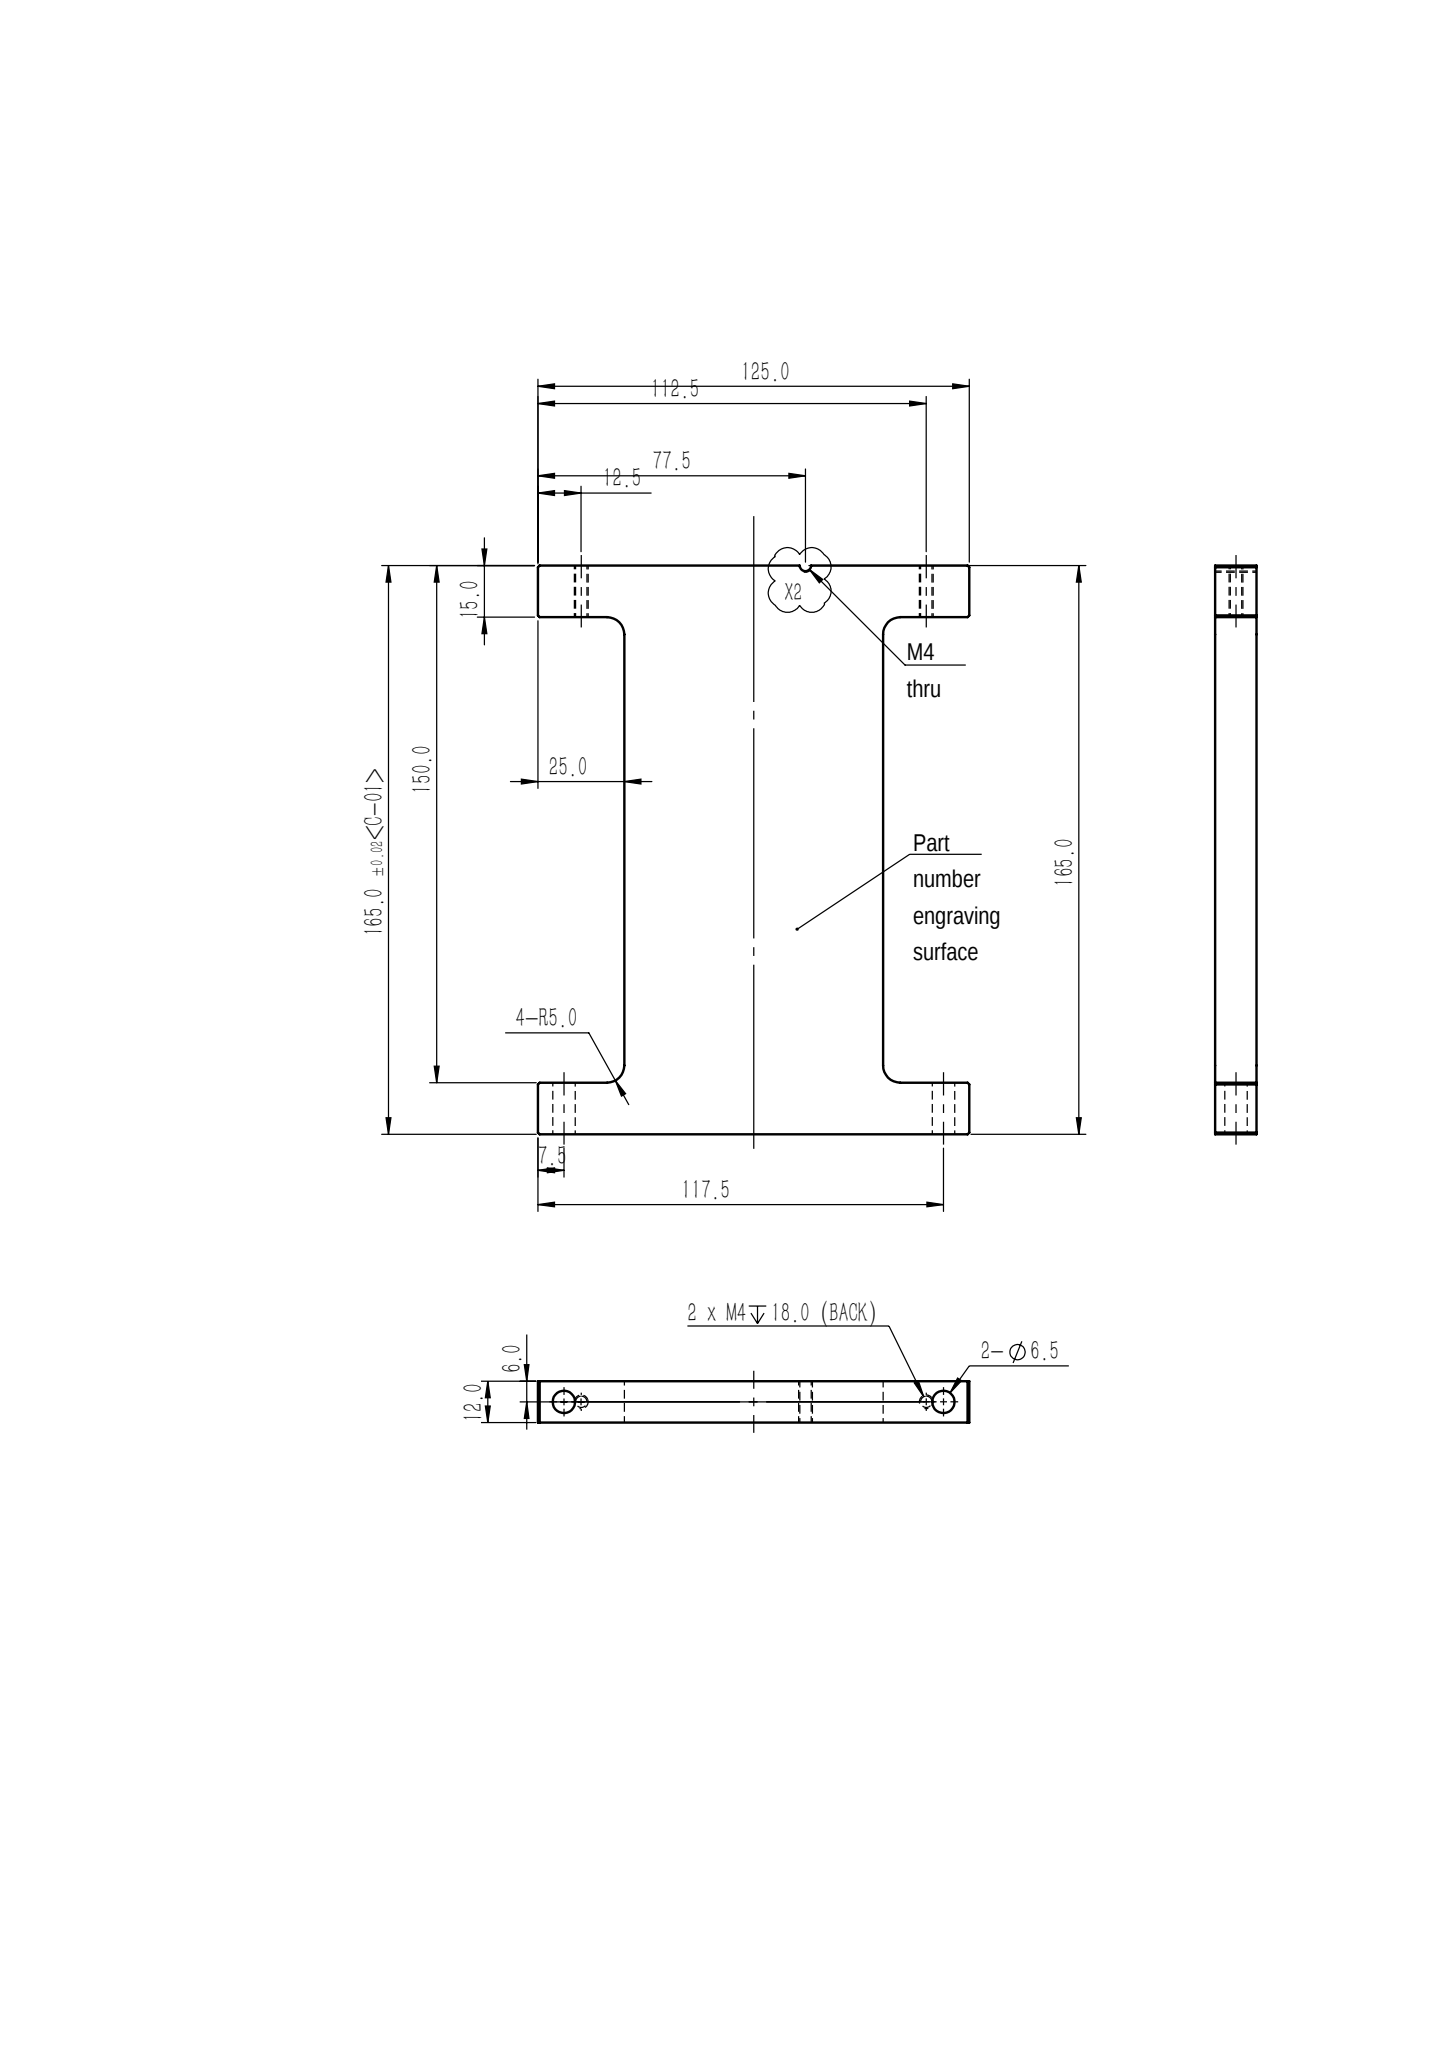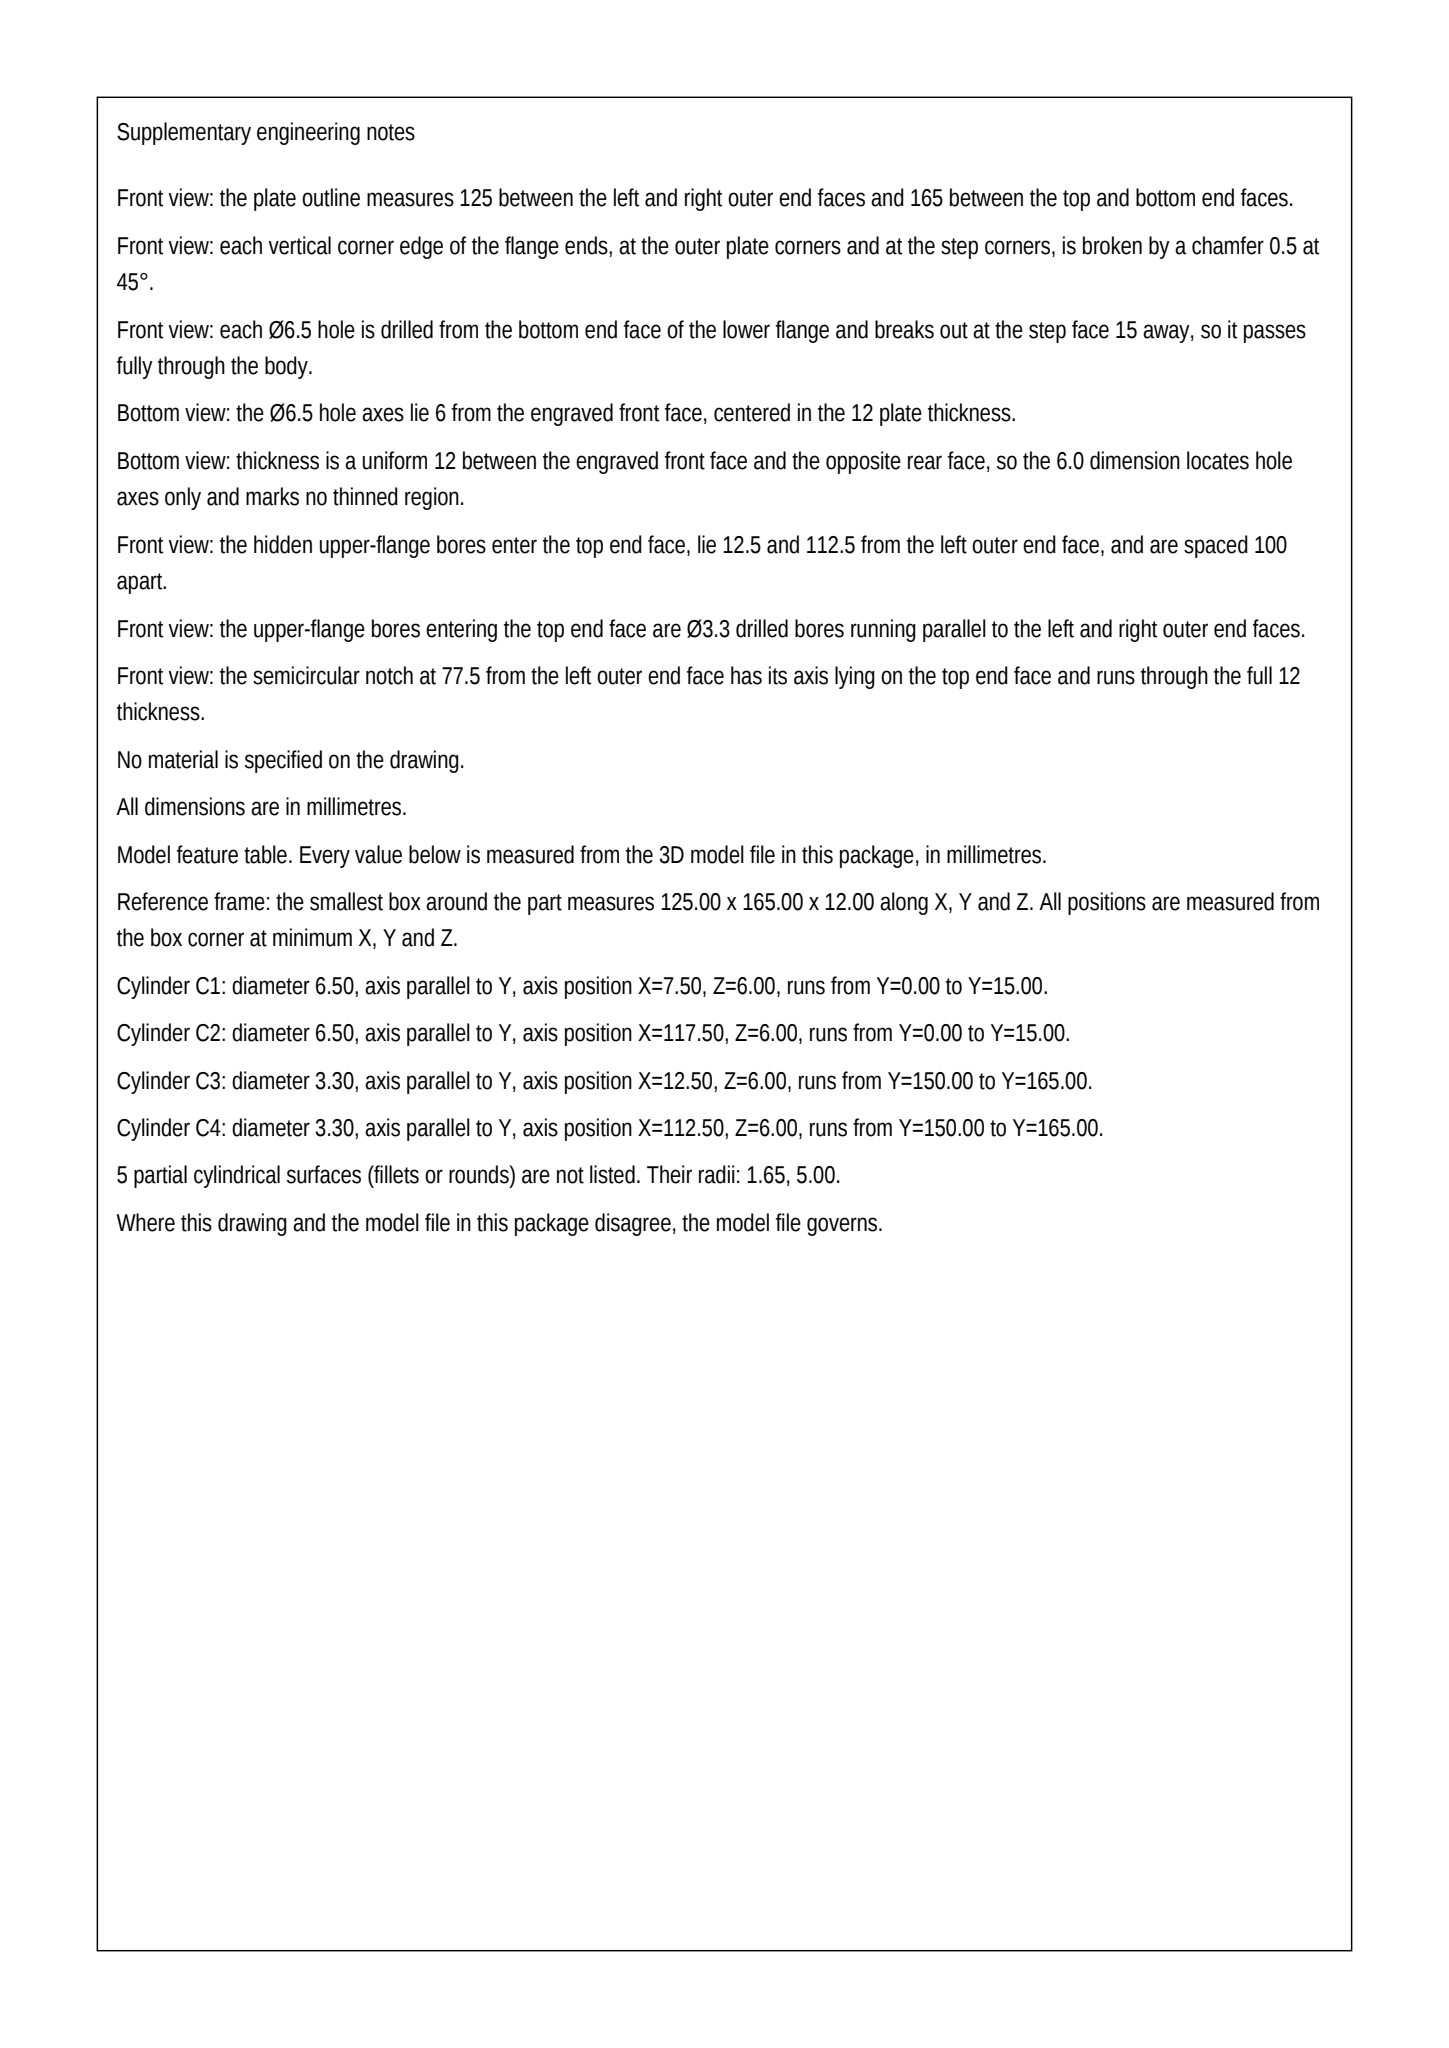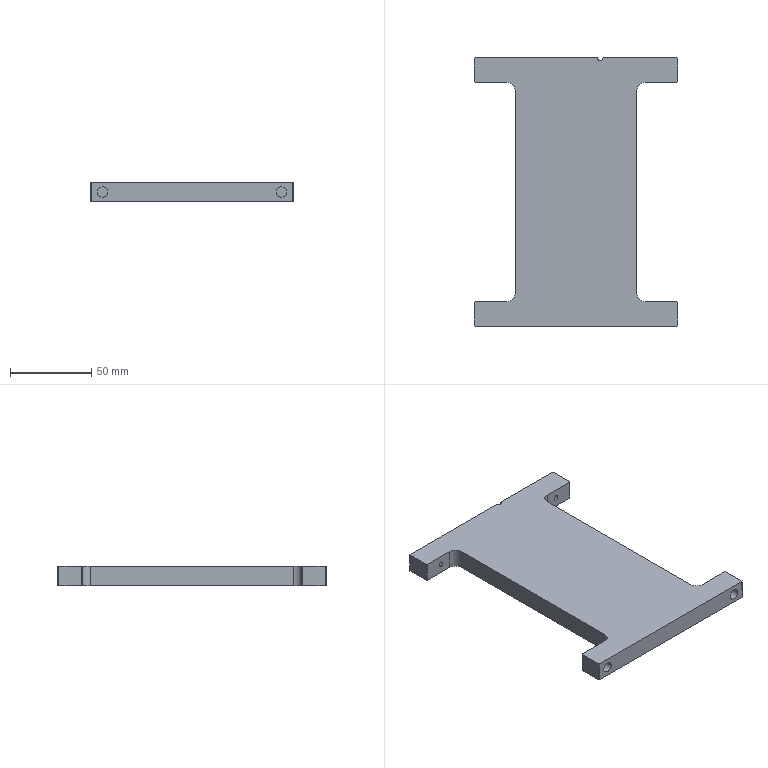Part | SolidWorks | mm | 1 solid | 36 faces | box 125 x 165 x 12 mm | volume 165442 mm3 | plane 23 | cylinder 13 | commonest cylinder face diameters 3.3 x5 6.5 x4 10 x4
build123d program:
from build123d import *

# Parameters (mm, degrees)
SKETCH1_W           = 125
SKETCH1_H           = 165
BOSS_EXTRUDE1_DEPTH = 12
SKETCH2_W           = 25
SKETCH2_H           = 135
CUT_EXTRUDE2_DEPTH  = 208.35
FILLET1_R           = 5
SKETCH3_R           = 3.25
CUT_EXTRUDE3_DEPTH  = 196.625
LPATTERN1_COUNT     = 2
LPATTERN1_PITCH     = 110
LPATTERN2_COUNT     = 2
LPATTERN2_PITCH     = 100
CHAMFER1_SIZE       = 0.5
M4_TAPPED_HOLE2_D   = 3.3


with BuildPart() as part:
    # Sketch1 → Boss-Extrude1 (new body)
    with BuildSketch(Plane.XY):
        with Locations((62.5, 82.5)):
            Rectangle(SKETCH1_W, SKETCH1_H)
    extrude(amount=BOSS_EXTRUDE1_DEPTH)

    # Sketch2 → Cut-Extrude2 (cut, through all)
    with BuildSketch(Plane.XY.offset(12)):
        with Locations((12.5, 82.5)):
            Rectangle(SKETCH2_W, SKETCH2_H)
        with Locations((112.5, 82.5)):
            Rectangle(SKETCH2_W, SKETCH2_H)
    extrude(amount=-CUT_EXTRUDE2_DEPTH, mode=Mode.SUBTRACT)

    # Fillet1
    fillet1_edges = [part.edges().sort_by_distance(p)[0] for p in [
        (25, 150, 6),
        (25, 15, 6),
        (100, 15, 6),
        (100, 150, 6),
    ]]
    fillet(fillet1_edges, radius=FILLET1_R)

    # Sketch3 → Cut-Extrude3 (cut, through all)
    with BuildSketch(Plane(origin=(0, 15, 0), x_dir=(1, 0, 0), z_dir=(0, 1, 0))):
        with Locations(Location((117.5, -6, 0), (0, 0, 180))):
            Circle(SKETCH3_R)
    cut_extrude3 = extrude(amount=-CUT_EXTRUDE3_DEPTH, mode=Mode.SUBTRACT)

    # LPattern1: Cut-Extrude3 ×2
    with Locations(*[(-i * LPATTERN1_PITCH, 0, 0) for i in range(1, LPATTERN1_COUNT)]):
        add(cut_extrude3, mode=Mode.SUBTRACT)

    # Sketch4 → M4 Tapped Hole1 (revolve, cut)
    with BuildSketch(Plane(origin=(112.5, 165, 6), x_dir=(0, 0, 1), z_dir=(1, 0, 0))):
        Polygon((0, 0), (0, 21.091), (1.65, 20.1), (1.65, 0), align=None)
    m4_tapped_hole1 = revolve(axis=Axis((112.5, 171.35, 6), (0, -1, 0)), mode=Mode.SUBTRACT)

    # LPattern2: M4 Tapped Hole1 ×2
    with Locations(*[(-i * LPATTERN2_PITCH, 0, 0) for i in range(1, LPATTERN2_COUNT)]):
        add(m4_tapped_hole1, mode=Mode.SUBTRACT)

    # Chamfer1
    chamfer1_edges = [part.edges().sort_by_distance(p)[0] for p in [
        (0, 15, 6),
        (0, 150, 6),
        (125, 150, 6),
        (125, 15, 6),
        (0, 165, 6),
        (125, 165, 6),
        (125, 0, 6),
        (0, 0, 6),
    ]]
    chamfer(chamfer1_edges, length=CHAMFER1_SIZE)

    # M4 Tapped Hole2 (through all)
    with Locations(Plane.XY.offset(12)):
        with Locations((77.5, 165)):
            Hole(M4_TAPPED_HOLE2_D / 2)


solid = part.part